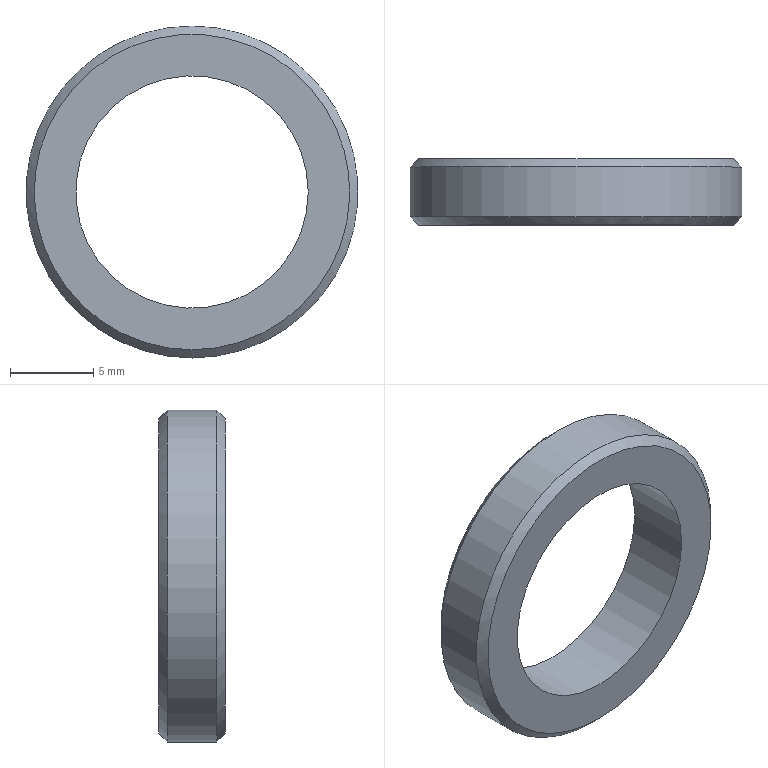Component | NX | NUT | 1 solid | 6 faces | box 20 x 4 x 20 mm | volume 625 mm3 | cylinder 2 | plane 2 | cone 2 | commonest cylinder face diameters 20 x1 14 x1
STEP:
#1=CARTESIAN_POINT('',(0.,0.,0.));
#2=DIRECTION('',(0.,0.,1.));
#3=DIRECTION('',(1.,0.,0.));
#4=AXIS2_PLACEMENT_3D('',#1,#2,#3);
#5=CARTESIAN_POINT('',(13.994,-99.616,-10.));
#6=VERTEX_POINT('',#5);
#7=CARTESIAN_POINT('',(13.994,-99.616,-0.));
#8=DIRECTION('',(0.,1.,0.));
#9=DIRECTION('',(0.,0.,-1.));
#10=AXIS2_PLACEMENT_3D('',#7,#8,#9);
#11=CIRCLE('',#10,10.);
#12=CARTESIAN_POINT('',(13.994,-100.116,-0.));
#13=DIRECTION('',(0.,1.,0.));
#14=DIRECTION('',(0.,0.,1.));
#15=AXIS2_PLACEMENT_3D('',#12,#13,#14);
#16=CYLINDRICAL_SURFACE('',#15,10.);
#17=CARTESIAN_POINT('',(3.142,0.5));
#18=DIRECTION('',(1.,0.));
#19=VECTOR('',#18,1.);
#20=LINE('',#17,#19);
#21=(GEOMETRIC_REPRESENTATION_CONTEXT(2)PARAMETRIC_REPRESENTATION_CONTEXT()REPRESENTATION_CONTEXT('',''));
#22=DEFINITIONAL_REPRESENTATION('',(#20),#21);
#23=PCURVE('',#16,#22);
#24=CARTESIAN_POINT('',(13.994,-100.116,-0.));
#25=DIRECTION('',(0.,1.,0.));
#26=DIRECTION('',(0.,0.,1.));
#27=AXIS2_PLACEMENT_3D('',#24,#25,#26);
#28=CONICAL_SURFACE('',#27,9.5,0.7854);
#29=CARTESIAN_POINT('',(3.142,0.5));
#30=DIRECTION('',(1.,0.));
#31=VECTOR('',#30,1.);
#32=LINE('',#29,#31);
#33=(GEOMETRIC_REPRESENTATION_CONTEXT(2)PARAMETRIC_REPRESENTATION_CONTEXT()REPRESENTATION_CONTEXT('',''));
#34=DEFINITIONAL_REPRESENTATION('',(#32),#33);
#35=PCURVE('',#28,#34);
#36=SURFACE_CURVE('',#11,(#23,#35),.PCURVE_S1.);
#37=EDGE_CURVE('',#6,#6,#36,.T.);
#38=ORIENTED_EDGE('',*,*,#37,.T.);
#39=CARTESIAN_POINT('',(13.994,-96.616,-10.));
#40=VERTEX_POINT('',#39);
#41=CARTESIAN_POINT('',(13.994,-99.616,-10.));
#42=CARTESIAN_POINT('',(13.994,-96.616,-10.));
#43=B_SPLINE_CURVE_WITH_KNOTS('',1,(#41,#42),.UNSPECIFIED.,.F.,.F.,(2,2),(0.5,3.5),.PIECEWISE_BEZIER_KNOTS.);
#44=CARTESIAN_POINT('',(9.425,0.));
#45=DIRECTION('',(0.,1.));
#46=VECTOR('',#45,1.);
#47=LINE('',#44,#46);
#48=(GEOMETRIC_REPRESENTATION_CONTEXT(2)PARAMETRIC_REPRESENTATION_CONTEXT()REPRESENTATION_CONTEXT('',''));
#49=DEFINITIONAL_REPRESENTATION('',(#47),#48);
#50=PCURVE('',#16,#49);
#51=CARTESIAN_POINT('',(3.142,0.));
#52=DIRECTION('',(0.,1.));
#53=VECTOR('',#52,1.);
#54=LINE('',#51,#53);
#55=(GEOMETRIC_REPRESENTATION_CONTEXT(2)PARAMETRIC_REPRESENTATION_CONTEXT()REPRESENTATION_CONTEXT('',''));
#56=DEFINITIONAL_REPRESENTATION('',(#54),#55);
#57=PCURVE('',#16,#56);
#58=SEAM_CURVE('',#43,(#50,#57),.PCURVE_S1.);
#59=EDGE_CURVE('',#6,#40,#58,.T.);
#60=ORIENTED_EDGE('',*,*,#59,.T.);
#61=CARTESIAN_POINT('',(13.994,-96.616,-0.));
#62=DIRECTION('',(0.,-1.,0.));
#63=DIRECTION('',(0.,0.,-1.));
#64=AXIS2_PLACEMENT_3D('',#61,#62,#63);
#65=CIRCLE('',#64,10.);
#66=CARTESIAN_POINT('',(9.425,3.5));
#67=DIRECTION('',(-1.,0.));
#68=VECTOR('',#67,1.);
#69=LINE('',#66,#68);
#70=(GEOMETRIC_REPRESENTATION_CONTEXT(2)PARAMETRIC_REPRESENTATION_CONTEXT()REPRESENTATION_CONTEXT('',''));
#71=DEFINITIONAL_REPRESENTATION('',(#69),#70);
#72=PCURVE('',#16,#71);
#73=CARTESIAN_POINT('',(13.994,-96.616,-0.));
#74=DIRECTION('',(0.,-1.,0.));
#75=DIRECTION('',(0.,0.,-1.));
#76=AXIS2_PLACEMENT_3D('',#73,#74,#75);
#77=CONICAL_SURFACE('',#76,10.,0.7854);
#78=CARTESIAN_POINT('',(0.,0.));
#79=DIRECTION('',(1.,0.));
#80=VECTOR('',#79,1.);
#81=LINE('',#78,#80);
#82=(GEOMETRIC_REPRESENTATION_CONTEXT(2)PARAMETRIC_REPRESENTATION_CONTEXT()REPRESENTATION_CONTEXT('',''));
#83=DEFINITIONAL_REPRESENTATION('',(#81),#82);
#84=PCURVE('',#77,#83);
#85=SURFACE_CURVE('',#65,(#72,#84),.PCURVE_S1.);
#86=EDGE_CURVE('',#40,#40,#85,.T.);
#87=ORIENTED_EDGE('',*,*,#86,.T.);
#88=ORIENTED_EDGE('',*,*,#59,.F.);
#89=EDGE_LOOP('',(#38,#60,#87,#88));
#90=FACE_BOUND('',#89,.T.);
#91=ADVANCED_FACE('',(#90),#16,.T.);
#92=CARTESIAN_POINT('',(20.994,-100.116,-0.));
#93=VERTEX_POINT('',#92);
#94=CARTESIAN_POINT('',(13.994,-100.116,-0.));
#95=DIRECTION('',(0.,-1.,0.));
#96=DIRECTION('',(1.,0.,-0.));
#97=AXIS2_PLACEMENT_3D('',#94,#95,#96);
#98=CIRCLE('',#97,7.);
#99=CARTESIAN_POINT('',(13.994,-100.116,-0.));
#100=DIRECTION('',(0.,1.,0.));
#101=DIRECTION('',(0.,0.,1.));
#102=AXIS2_PLACEMENT_3D('',#99,#100,#101);
#103=CYLINDRICAL_SURFACE('',#102,7.);
#104=CARTESIAN_POINT('',(7.854,0.));
#105=DIRECTION('',(-1.,0.));
#106=VECTOR('',#105,1.);
#107=LINE('',#104,#106);
#108=(GEOMETRIC_REPRESENTATION_CONTEXT(2)PARAMETRIC_REPRESENTATION_CONTEXT()REPRESENTATION_CONTEXT('',''));
#109=DEFINITIONAL_REPRESENTATION('',(#107),#108);
#110=PCURVE('',#103,#109);
#111=CARTESIAN_POINT('',(13.994,-100.116,-0.));
#112=DIRECTION('',(0.,-1.,0.));
#113=DIRECTION('',(0.,0.,-1.));
#114=AXIS2_PLACEMENT_3D('',#111,#112,#113);
#115=PLANE('',#114);
#116=CARTESIAN_POINT('',(0.,0.));
#117=DIRECTION('',(0.,1.));
#118=AXIS2_PLACEMENT_2D('',#116,#117);
#119=CIRCLE('',#118,7.);
#120=(GEOMETRIC_REPRESENTATION_CONTEXT(2)PARAMETRIC_REPRESENTATION_CONTEXT()REPRESENTATION_CONTEXT('',''));
#121=DEFINITIONAL_REPRESENTATION('',(#119),#120);
#122=PCURVE('',#115,#121);
#123=SURFACE_CURVE('',#98,(#110,#122),.PCURVE_S1.);
#124=EDGE_CURVE('',#93,#93,#123,.T.);
#125=ORIENTED_EDGE('',*,*,#124,.F.);
#126=CARTESIAN_POINT('',(20.994,-96.116,-0.));
#127=VERTEX_POINT('',#126);
#128=CARTESIAN_POINT('',(20.994,-100.116,-0.));
#129=CARTESIAN_POINT('',(20.994,-96.116,-0.));
#130=B_SPLINE_CURVE_WITH_KNOTS('',1,(#128,#129),.UNSPECIFIED.,.F.,.F.,(2,2),(0.,4.),.PIECEWISE_BEZIER_KNOTS.);
#131=CARTESIAN_POINT('',(7.854,0.));
#132=DIRECTION('',(0.,1.));
#133=VECTOR('',#132,1.);
#134=LINE('',#131,#133);
#135=(GEOMETRIC_REPRESENTATION_CONTEXT(2)PARAMETRIC_REPRESENTATION_CONTEXT()REPRESENTATION_CONTEXT('',''));
#136=DEFINITIONAL_REPRESENTATION('',(#134),#135);
#137=PCURVE('',#103,#136);
#138=CARTESIAN_POINT('',(1.571,0.));
#139=DIRECTION('',(0.,1.));
#140=VECTOR('',#139,1.);
#141=LINE('',#138,#140);
#142=(GEOMETRIC_REPRESENTATION_CONTEXT(2)PARAMETRIC_REPRESENTATION_CONTEXT()REPRESENTATION_CONTEXT('',''));
#143=DEFINITIONAL_REPRESENTATION('',(#141),#142);
#144=PCURVE('',#103,#143);
#145=SEAM_CURVE('',#130,(#137,#144),.PCURVE_S1.);
#146=EDGE_CURVE('',#93,#127,#145,.T.);
#147=ORIENTED_EDGE('',*,*,#146,.T.);
#148=CARTESIAN_POINT('',(13.994,-96.116,-0.));
#149=DIRECTION('',(0.,-1.,0.));
#150=DIRECTION('',(1.,0.,-0.));
#151=AXIS2_PLACEMENT_3D('',#148,#149,#150);
#152=CIRCLE('',#151,7.);
#153=CARTESIAN_POINT('',(7.854,4.));
#154=DIRECTION('',(-1.,0.));
#155=VECTOR('',#154,1.);
#156=LINE('',#153,#155);
#157=(GEOMETRIC_REPRESENTATION_CONTEXT(2)PARAMETRIC_REPRESENTATION_CONTEXT()REPRESENTATION_CONTEXT('',''));
#158=DEFINITIONAL_REPRESENTATION('',(#156),#157);
#159=PCURVE('',#103,#158);
#160=CARTESIAN_POINT('',(13.994,-96.116,-0.));
#161=DIRECTION('',(0.,-1.,0.));
#162=DIRECTION('',(0.,0.,-1.));
#163=AXIS2_PLACEMENT_3D('',#160,#161,#162);
#164=PLANE('',#163);
#165=CARTESIAN_POINT('',(0.,0.));
#166=DIRECTION('',(0.,1.));
#167=AXIS2_PLACEMENT_2D('',#165,#166);
#168=CIRCLE('',#167,7.);
#169=(GEOMETRIC_REPRESENTATION_CONTEXT(2)PARAMETRIC_REPRESENTATION_CONTEXT()REPRESENTATION_CONTEXT('',''));
#170=DEFINITIONAL_REPRESENTATION('',(#168),#169);
#171=PCURVE('',#164,#170);
#172=SURFACE_CURVE('',#152,(#159,#171),.PCURVE_S1.);
#173=EDGE_CURVE('',#127,#127,#172,.T.);
#174=ORIENTED_EDGE('',*,*,#173,.T.);
#175=ORIENTED_EDGE('',*,*,#146,.F.);
#176=EDGE_LOOP('',(#125,#147,#174,#175));
#177=FACE_BOUND('',#176,.F.);
#178=ADVANCED_FACE('',(#177),#103,.F.);
#179=CARTESIAN_POINT('',(13.994,-100.116,-9.5));
#180=VERTEX_POINT('',#179);
#181=CARTESIAN_POINT('',(13.994,-100.116,-0.));
#182=DIRECTION('',(0.,-1.,0.));
#183=DIRECTION('',(0.,0.,-1.));
#184=AXIS2_PLACEMENT_3D('',#181,#182,#183);
#185=CIRCLE('',#184,9.5);
#186=CARTESIAN_POINT('',(0.,0.));
#187=DIRECTION('',(1.,0.));
#188=AXIS2_PLACEMENT_2D('',#186,#187);
#189=CIRCLE('',#188,9.5);
#190=(GEOMETRIC_REPRESENTATION_CONTEXT(2)PARAMETRIC_REPRESENTATION_CONTEXT()REPRESENTATION_CONTEXT('',''));
#191=DEFINITIONAL_REPRESENTATION('',(#189),#190);
#192=PCURVE('',#115,#191);
#193=CARTESIAN_POINT('',(9.425,0.));
#194=DIRECTION('',(-1.,0.));
#195=VECTOR('',#194,1.);
#196=LINE('',#193,#195);
#197=(GEOMETRIC_REPRESENTATION_CONTEXT(2)PARAMETRIC_REPRESENTATION_CONTEXT()REPRESENTATION_CONTEXT('',''));
#198=DEFINITIONAL_REPRESENTATION('',(#196),#197);
#199=PCURVE('',#28,#198);
#200=SURFACE_CURVE('',#185,(#192,#199),.PCURVE_S1.);
#201=EDGE_CURVE('',#180,#180,#200,.T.);
#202=ORIENTED_EDGE('',*,*,#201,.T.);
#203=EDGE_LOOP('',(#202));
#204=FACE_BOUND('',#203,.T.);
#205=ORIENTED_EDGE('',*,*,#124,.F.);
#206=EDGE_LOOP('',(#205));
#207=FACE_BOUND('',#206,.T.);
#208=ADVANCED_FACE('',(#204,#207),#115,.T.);
#209=CARTESIAN_POINT('',(13.994,-96.116,-9.5));
#210=VERTEX_POINT('',#209);
#211=CARTESIAN_POINT('',(13.994,-96.116,-0.));
#212=DIRECTION('',(0.,1.,0.));
#213=DIRECTION('',(0.,0.,-1.));
#214=AXIS2_PLACEMENT_3D('',#211,#212,#213);
#215=CIRCLE('',#214,9.5);
#216=CARTESIAN_POINT('',(9.5,0.));
#217=CARTESIAN_POINT('',(9.5,-16.454));
#218=CARTESIAN_POINT('',(-4.75,-8.227));
#219=CARTESIAN_POINT('',(-19.,-0.));
#220=CARTESIAN_POINT('',(-4.75,8.227));
#221=CARTESIAN_POINT('',(9.5,16.454));
#222=CARTESIAN_POINT('',(9.5,0.));
#223=(BOUNDED_CURVE()B_SPLINE_CURVE(2,(#216,#217,#218,#219,#220,#221,#222),.UNSPECIFIED.,.T.,.F.)B_SPLINE_CURVE_WITH_KNOTS((1,2,2,2,2,1),(-2.094,0.,2.094,4.189,6.283,8.378),.UNSPECIFIED.)CURVE()GEOMETRIC_REPRESENTATION_ITEM()RATIONAL_B_SPLINE_CURVE((1.,0.5,1.,0.5,1.,0.5,1.))REPRESENTATION_ITEM(''));
#224=(GEOMETRIC_REPRESENTATION_CONTEXT(2)PARAMETRIC_REPRESENTATION_CONTEXT()REPRESENTATION_CONTEXT('',''));
#225=DEFINITIONAL_REPRESENTATION('',(#223),#224);
#226=PCURVE('',#164,#225);
#227=CARTESIAN_POINT('',(6.283,-0.5));
#228=DIRECTION('',(-1.,0.));
#229=VECTOR('',#228,1.);
#230=LINE('',#227,#229);
#231=(GEOMETRIC_REPRESENTATION_CONTEXT(2)PARAMETRIC_REPRESENTATION_CONTEXT()REPRESENTATION_CONTEXT('',''));
#232=DEFINITIONAL_REPRESENTATION('',(#230),#231);
#233=PCURVE('',#77,#232);
#234=SURFACE_CURVE('',#215,(#226,#233),.PCURVE_S1.);
#235=EDGE_CURVE('',#210,#210,#234,.T.);
#236=ORIENTED_EDGE('',*,*,#235,.T.);
#237=EDGE_LOOP('',(#236));
#238=FACE_BOUND('',#237,.T.);
#239=ORIENTED_EDGE('',*,*,#173,.T.);
#240=EDGE_LOOP('',(#239));
#241=FACE_BOUND('',#240,.T.);
#242=ADVANCED_FACE('',(#238,#241),#164,.F.);
#243=ORIENTED_EDGE('',*,*,#37,.F.);
#244=CARTESIAN_POINT('',(13.994,-100.116,-9.5));
#245=CARTESIAN_POINT('',(13.994,-99.616,-10.));
#246=B_SPLINE_CURVE_WITH_KNOTS('',1,(#244,#245),.UNSPECIFIED.,.F.,.F.,(2,2),(0.,0.7071),.PIECEWISE_BEZIER_KNOTS.);
#247=CARTESIAN_POINT('',(3.142,0.));
#248=DIRECTION('',(0.,1.));
#249=VECTOR('',#248,1.);
#250=LINE('',#247,#249);
#251=(GEOMETRIC_REPRESENTATION_CONTEXT(2)PARAMETRIC_REPRESENTATION_CONTEXT()REPRESENTATION_CONTEXT('',''));
#252=DEFINITIONAL_REPRESENTATION('',(#250),#251);
#253=PCURVE('',#28,#252);
#254=CARTESIAN_POINT('',(9.425,0.));
#255=DIRECTION('',(0.,1.));
#256=VECTOR('',#255,1.);
#257=LINE('',#254,#256);
#258=(GEOMETRIC_REPRESENTATION_CONTEXT(2)PARAMETRIC_REPRESENTATION_CONTEXT()REPRESENTATION_CONTEXT('',''));
#259=DEFINITIONAL_REPRESENTATION('',(#257),#258);
#260=PCURVE('',#28,#259);
#261=SEAM_CURVE('',#246,(#253,#260),.PCURVE_S1.);
#262=EDGE_CURVE('',#180,#6,#261,.T.);
#263=ORIENTED_EDGE('',*,*,#262,.F.);
#264=ORIENTED_EDGE('',*,*,#201,.F.);
#265=ORIENTED_EDGE('',*,*,#262,.T.);
#266=EDGE_LOOP('',(#243,#263,#264,#265));
#267=FACE_BOUND('',#266,.T.);
#268=ADVANCED_FACE('',(#267),#28,.T.);
#269=ORIENTED_EDGE('',*,*,#235,.F.);
#270=CARTESIAN_POINT('',(13.994,-96.116,-9.5));
#271=CARTESIAN_POINT('',(13.994,-96.616,-10.));
#272=B_SPLINE_CURVE_WITH_KNOTS('',1,(#270,#271),.UNSPECIFIED.,.F.,.F.,(2,2),(-0.7071,0.),.PIECEWISE_BEZIER_KNOTS.);
#273=CARTESIAN_POINT('',(6.283,0.));
#274=DIRECTION('',(0.,1.));
#275=VECTOR('',#274,1.);
#276=LINE('',#273,#275);
#277=(GEOMETRIC_REPRESENTATION_CONTEXT(2)PARAMETRIC_REPRESENTATION_CONTEXT()REPRESENTATION_CONTEXT('',''));
#278=DEFINITIONAL_REPRESENTATION('',(#276),#277);
#279=PCURVE('',#77,#278);
#280=CARTESIAN_POINT('',(0.,0.));
#281=DIRECTION('',(0.,1.));
#282=VECTOR('',#281,1.);
#283=LINE('',#280,#282);
#284=(GEOMETRIC_REPRESENTATION_CONTEXT(2)PARAMETRIC_REPRESENTATION_CONTEXT()REPRESENTATION_CONTEXT('',''));
#285=DEFINITIONAL_REPRESENTATION('',(#283),#284);
#286=PCURVE('',#77,#285);
#287=SEAM_CURVE('',#272,(#279,#286),.PCURVE_S1.);
#288=EDGE_CURVE('',#210,#40,#287,.T.);
#289=ORIENTED_EDGE('',*,*,#288,.T.);
#290=ORIENTED_EDGE('',*,*,#86,.F.);
#291=ORIENTED_EDGE('',*,*,#288,.F.);
#292=EDGE_LOOP('',(#269,#289,#290,#291));
#293=FACE_BOUND('',#292,.T.);
#294=ADVANCED_FACE('',(#293),#77,.T.);
#295=CLOSED_SHELL('',(#91,#178,#208,#242,#268,#294));
#296=MANIFOLD_SOLID_BREP('',#295);
#297=(LENGTH_UNIT()NAMED_UNIT(*)SI_UNIT(.MILLI.,.METRE.));
#298=UNCERTAINTY_MEASURE_WITH_UNIT(LENGTH_MEASURE(0.00001),#297,'','');
#299=(NAMED_UNIT(*)PLANE_ANGLE_UNIT()SI_UNIT($,.RADIAN.));
#300=(NAMED_UNIT(*)SI_UNIT($,.STERADIAN.)SOLID_ANGLE_UNIT());
#301=(GEOMETRIC_REPRESENTATION_CONTEXT(3)GLOBAL_UNCERTAINTY_ASSIGNED_CONTEXT((#298))GLOBAL_UNIT_ASSIGNED_CONTEXT((#297,#299,#300))REPRESENTATION_CONTEXT('',''));
#302=ADVANCED_BREP_SHAPE_REPRESENTATION('',(#4,#296),#301);